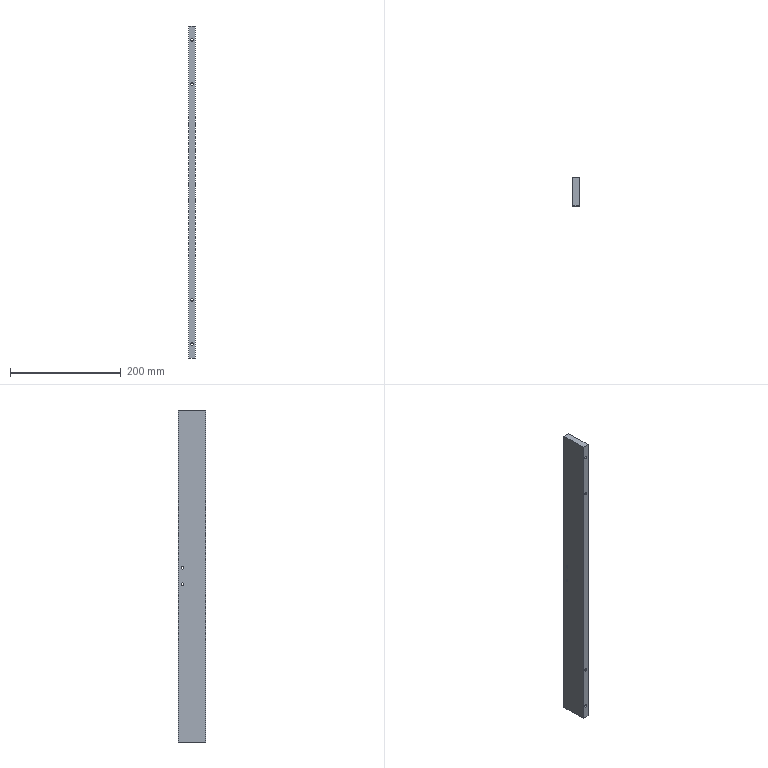Component | SolidWorks | SupportPlate-2 | 1 solid | 18 faces | box 12 x 50 x 600 mm | volume 355602 mm3 | cylinder 12 | plane 6 | commonest cylinder face diameters 5 x12
build123d program:
from build123d import *

# Parameters (mm, degrees)
SKETCH1_W             = 12
SKETCH1_H             = 50
EXTRUDE1_DEPTH        = 600
M6_TAPPED_HOLE1_D     = 5
M6_TAPPED_HOLE2_D     = 5
M6_TAPPED_HOLE2_DEPTH = 15
M6_TAPPED_HOLE2_TIP   = 1.502


with BuildPart() as part:
    # Sketch1 → Extrude1 (new body)
    with BuildSketch(Plane.XY):
        with Locations((49.859, -11.771)):
            Rectangle(SKETCH1_W, SKETCH1_H)
    extrude(amount=EXTRUDE1_DEPTH)

    # M6 Tapped Hole1 (through all)
    with Locations(Plane(origin=(0, 13.229, 0), x_dir=(-1, 0, 0), z_dir=(0, 1, 0))):
        with Locations((-49.859, 25), (-49.859, 105), (-49.859, 575), (-49.859, 495)):
            Hole(M6_TAPPED_HOLE1_D / 2)

    # M6 Tapped Hole2
    with Locations(Plane.ZY.offset(-43.859)):
        with Locations((315, 5.229), (285, 5.229)):
            Hole(M6_TAPPED_HOLE2_D / 2, depth=M6_TAPPED_HOLE2_DEPTH)
            with Locations((0, 0, -(M6_TAPPED_HOLE2_DEPTH + M6_TAPPED_HOLE2_TIP / 2))):  # 118° drill point
                Cone(0, M6_TAPPED_HOLE2_D / 2, M6_TAPPED_HOLE2_TIP, mode=Mode.SUBTRACT)


solid = part.part

# Placed as in the assembly
solid = solid.moved(Location((4.357, 407.754, -296), (0, 0, 0)))
STEP:
#1=COLOUR_RGB('',0.7922,0.8196,0.9333);
#2=FILL_AREA_STYLE_COLOUR('',#1);
#3=FILL_AREA_STYLE('',(#2));
#4=SURFACE_STYLE_FILL_AREA(#3);
#5=SURFACE_SIDE_STYLE('',(#4));
#6=SURFACE_STYLE_USAGE(.BOTH.,#5);
#7=PRESENTATION_STYLE_ASSIGNMENT((#6));
#8=CARTESIAN_POINT('',(2.371,16.259,0.6496));
#9=VERTEX_POINT('',#8);
#10=CARTESIAN_POINT('',(2.371,16.259,0.8465));
#11=VERTEX_POINT('',#10);
#12=CARTESIAN_POINT('',(2.371,16.259,0.748));
#13=DIRECTION('',(-1.,-0.,0.));
#14=DIRECTION('',(0.,-1.,0.));
#15=AXIS2_PLACEMENT_3D('',#12,#13,#14);
#16=CIRCLE('',#15,0.09843);
#17=EDGE_CURVE('',#9,#11,#16,.T.);
#18=ORIENTED_EDGE('',*,*,#17,.F.);
#19=CARTESIAN_POINT('',(1.898,16.259,0.6496));
#20=VERTEX_POINT('',#19);
#21=CARTESIAN_POINT('',(1.898,16.259,0.6496));
#22=DIRECTION('',(-1.,0.,0.));
#23=VECTOR('',#22,39.37);
#24=LINE('',#21,#23);
#25=EDGE_CURVE('',#9,#20,#24,.T.);
#26=ORIENTED_EDGE('',*,*,#25,.T.);
#27=CARTESIAN_POINT('',(1.898,16.259,0.8465));
#28=VERTEX_POINT('',#27);
#29=CARTESIAN_POINT('',(1.898,16.259,0.748));
#30=DIRECTION('',(-1.,0.,0.));
#31=DIRECTION('',(0.,0.,1.));
#32=AXIS2_PLACEMENT_3D('',#29,#30,#31);
#33=CIRCLE('',#32,0.09843);
#34=EDGE_CURVE('',#20,#28,#33,.T.);
#35=ORIENTED_EDGE('',*,*,#34,.T.);
#36=CARTESIAN_POINT('',(1.898,16.259,0.8465));
#37=DIRECTION('',(-1.,0.,0.));
#38=VECTOR('',#37,39.37);
#39=LINE('',#36,#38);
#40=EDGE_CURVE('',#11,#28,#39,.T.);
#41=ORIENTED_EDGE('',*,*,#40,.F.);
#42=EDGE_LOOP('',(#18,#26,#35,#41));
#43=FACE_OUTER_BOUND('',#42,.T.);
#44=CARTESIAN_POINT('',(1.898,16.259,0.748));
#45=DIRECTION('',(-1.,0.,0.));
#46=DIRECTION('',(0.,0.,1.));
#47=AXIS2_PLACEMENT_3D('',#44,#45,#46);
#48=CYLINDRICAL_SURFACE('',#47,0.09843);
#49=ADVANCED_FACE('',(#43),#48,.F.);
#50=CARTESIAN_POINT('',(2.371,16.259,-0.5315));
#51=VERTEX_POINT('',#50);
#52=CARTESIAN_POINT('',(2.371,16.259,-0.3346));
#53=VERTEX_POINT('',#52);
#54=CARTESIAN_POINT('',(2.371,16.259,-0.4331));
#55=DIRECTION('',(-1.,-0.,0.));
#56=DIRECTION('',(0.,-1.,0.));
#57=AXIS2_PLACEMENT_3D('',#54,#55,#56);
#58=CIRCLE('',#57,0.09843);
#59=EDGE_CURVE('',#51,#53,#58,.T.);
#60=ORIENTED_EDGE('',*,*,#59,.F.);
#61=CARTESIAN_POINT('',(1.898,16.259,-0.5315));
#62=VERTEX_POINT('',#61);
#63=CARTESIAN_POINT('',(1.898,16.259,-0.5315));
#64=DIRECTION('',(-1.,0.,0.));
#65=VECTOR('',#64,39.37);
#66=LINE('',#63,#65);
#67=EDGE_CURVE('',#51,#62,#66,.T.);
#68=ORIENTED_EDGE('',*,*,#67,.T.);
#69=CARTESIAN_POINT('',(1.898,16.259,-0.3346));
#70=VERTEX_POINT('',#69);
#71=CARTESIAN_POINT('',(1.898,16.259,-0.4331));
#72=DIRECTION('',(-1.,0.,0.));
#73=DIRECTION('',(0.,0.,1.));
#74=AXIS2_PLACEMENT_3D('',#71,#72,#73);
#75=CIRCLE('',#74,0.09843);
#76=EDGE_CURVE('',#62,#70,#75,.T.);
#77=ORIENTED_EDGE('',*,*,#76,.T.);
#78=CARTESIAN_POINT('',(1.898,16.259,-0.3346));
#79=DIRECTION('',(-1.,0.,0.));
#80=VECTOR('',#79,39.37);
#81=LINE('',#78,#80);
#82=EDGE_CURVE('',#53,#70,#81,.T.);
#83=ORIENTED_EDGE('',*,*,#82,.F.);
#84=EDGE_LOOP('',(#60,#68,#77,#83));
#85=FACE_OUTER_BOUND('',#84,.T.);
#86=CARTESIAN_POINT('',(1.898,16.259,-0.4331));
#87=DIRECTION('',(-1.,0.,0.));
#88=DIRECTION('',(0.,0.,1.));
#89=AXIS2_PLACEMENT_3D('',#86,#87,#88);
#90=CYLINDRICAL_SURFACE('',#89,0.09843);
#91=ADVANCED_FACE('',(#85),#90,.F.);
#92=CARTESIAN_POINT('',(2.134,14.606,-10.768));
#93=VERTEX_POINT('',#92);
#94=CARTESIAN_POINT('',(2.134,14.606,-10.571));
#95=VERTEX_POINT('',#94);
#96=CARTESIAN_POINT('',(2.134,14.606,-10.669));
#97=DIRECTION('',(0.,1.,0.));
#98=DIRECTION('',(0.,0.,1.));
#99=AXIS2_PLACEMENT_3D('',#96,#97,#98);
#100=CIRCLE('',#99,0.09843);
#101=EDGE_CURVE('',#93,#95,#100,.T.);
#102=ORIENTED_EDGE('',*,*,#101,.F.);
#103=CARTESIAN_POINT('',(2.134,16.574,-10.768));
#104=VERTEX_POINT('',#103);
#105=CARTESIAN_POINT('',(2.134,16.574,-10.768));
#106=DIRECTION('',(0.,1.,0.));
#107=VECTOR('',#106,39.37);
#108=LINE('',#105,#107);
#109=EDGE_CURVE('',#93,#104,#108,.T.);
#110=ORIENTED_EDGE('',*,*,#109,.T.);
#111=CARTESIAN_POINT('',(2.134,16.574,-10.571));
#112=VERTEX_POINT('',#111);
#113=CARTESIAN_POINT('',(2.134,16.574,-10.669));
#114=DIRECTION('',(0.,1.,0.));
#115=DIRECTION('',(0.,0.,1.));
#116=AXIS2_PLACEMENT_3D('',#113,#114,#115);
#117=CIRCLE('',#116,0.09843);
#118=EDGE_CURVE('',#104,#112,#117,.T.);
#119=ORIENTED_EDGE('',*,*,#118,.T.);
#120=CARTESIAN_POINT('',(2.134,16.574,-10.571));
#121=DIRECTION('',(0.,1.,0.));
#122=VECTOR('',#121,39.37);
#123=LINE('',#120,#122);
#124=EDGE_CURVE('',#95,#112,#123,.T.);
#125=ORIENTED_EDGE('',*,*,#124,.F.);
#126=EDGE_LOOP('',(#102,#110,#119,#125));
#127=FACE_OUTER_BOUND('',#126,.T.);
#128=CARTESIAN_POINT('',(2.134,16.574,-10.669));
#129=DIRECTION('',(0.,1.,0.));
#130=DIRECTION('',(0.,0.,1.));
#131=AXIS2_PLACEMENT_3D('',#128,#129,#130);
#132=CYLINDRICAL_SURFACE('',#131,0.09843);
#133=ADVANCED_FACE('',(#127),#132,.F.);
#134=CARTESIAN_POINT('',(2.134,14.606,-7.618));
#135=VERTEX_POINT('',#134);
#136=CARTESIAN_POINT('',(2.134,14.606,-7.421));
#137=VERTEX_POINT('',#136);
#138=CARTESIAN_POINT('',(2.134,14.606,-7.52));
#139=DIRECTION('',(0.,1.,0.));
#140=DIRECTION('',(0.,0.,1.));
#141=AXIS2_PLACEMENT_3D('',#138,#139,#140);
#142=CIRCLE('',#141,0.09843);
#143=EDGE_CURVE('',#135,#137,#142,.T.);
#144=ORIENTED_EDGE('',*,*,#143,.F.);
#145=CARTESIAN_POINT('',(2.134,16.574,-7.618));
#146=VERTEX_POINT('',#145);
#147=CARTESIAN_POINT('',(2.134,16.574,-7.618));
#148=DIRECTION('',(0.,1.,0.));
#149=VECTOR('',#148,39.37);
#150=LINE('',#147,#149);
#151=EDGE_CURVE('',#135,#146,#150,.T.);
#152=ORIENTED_EDGE('',*,*,#151,.T.);
#153=CARTESIAN_POINT('',(2.134,16.574,-7.421));
#154=VERTEX_POINT('',#153);
#155=CARTESIAN_POINT('',(2.134,16.574,-7.52));
#156=DIRECTION('',(0.,1.,0.));
#157=DIRECTION('',(0.,0.,1.));
#158=AXIS2_PLACEMENT_3D('',#155,#156,#157);
#159=CIRCLE('',#158,0.09843);
#160=EDGE_CURVE('',#146,#154,#159,.T.);
#161=ORIENTED_EDGE('',*,*,#160,.T.);
#162=CARTESIAN_POINT('',(2.134,16.574,-7.421));
#163=DIRECTION('',(0.,1.,0.));
#164=VECTOR('',#163,39.37);
#165=LINE('',#162,#164);
#166=EDGE_CURVE('',#137,#154,#165,.T.);
#167=ORIENTED_EDGE('',*,*,#166,.F.);
#168=EDGE_LOOP('',(#144,#152,#161,#167));
#169=FACE_OUTER_BOUND('',#168,.T.);
#170=CARTESIAN_POINT('',(2.134,16.574,-7.52));
#171=DIRECTION('',(0.,1.,0.));
#172=DIRECTION('',(0.,0.,1.));
#173=AXIS2_PLACEMENT_3D('',#170,#171,#172);
#174=CYLINDRICAL_SURFACE('',#173,0.09843);
#175=ADVANCED_FACE('',(#169),#174,.F.);
#176=CARTESIAN_POINT('',(2.134,14.606,10.886));
#177=VERTEX_POINT('',#176);
#178=CARTESIAN_POINT('',(2.134,14.606,11.083));
#179=VERTEX_POINT('',#178);
#180=CARTESIAN_POINT('',(2.134,14.606,10.984));
#181=DIRECTION('',(0.,1.,0.));
#182=DIRECTION('',(0.,0.,1.));
#183=AXIS2_PLACEMENT_3D('',#180,#181,#182);
#184=CIRCLE('',#183,0.09843);
#185=EDGE_CURVE('',#177,#179,#184,.T.);
#186=ORIENTED_EDGE('',*,*,#185,.F.);
#187=CARTESIAN_POINT('',(2.134,16.574,10.886));
#188=VERTEX_POINT('',#187);
#189=CARTESIAN_POINT('',(2.134,16.574,10.886));
#190=DIRECTION('',(0.,1.,0.));
#191=VECTOR('',#190,39.37);
#192=LINE('',#189,#191);
#193=EDGE_CURVE('',#177,#188,#192,.T.);
#194=ORIENTED_EDGE('',*,*,#193,.T.);
#195=CARTESIAN_POINT('',(2.134,16.574,11.083));
#196=VERTEX_POINT('',#195);
#197=CARTESIAN_POINT('',(2.134,16.574,10.984));
#198=DIRECTION('',(0.,1.,0.));
#199=DIRECTION('',(0.,0.,1.));
#200=AXIS2_PLACEMENT_3D('',#197,#198,#199);
#201=CIRCLE('',#200,0.09843);
#202=EDGE_CURVE('',#188,#196,#201,.T.);
#203=ORIENTED_EDGE('',*,*,#202,.T.);
#204=CARTESIAN_POINT('',(2.134,16.574,11.083));
#205=DIRECTION('',(0.,1.,0.));
#206=VECTOR('',#205,39.37);
#207=LINE('',#204,#206);
#208=EDGE_CURVE('',#179,#196,#207,.T.);
#209=ORIENTED_EDGE('',*,*,#208,.F.);
#210=EDGE_LOOP('',(#186,#194,#203,#209));
#211=FACE_OUTER_BOUND('',#210,.T.);
#212=CARTESIAN_POINT('',(2.134,16.574,10.984));
#213=DIRECTION('',(0.,1.,0.));
#214=DIRECTION('',(0.,0.,1.));
#215=AXIS2_PLACEMENT_3D('',#212,#213,#214);
#216=CYLINDRICAL_SURFACE('',#215,0.09843);
#217=ADVANCED_FACE('',(#211),#216,.F.);
#218=CARTESIAN_POINT('',(2.134,14.606,7.736));
#219=VERTEX_POINT('',#218);
#220=CARTESIAN_POINT('',(2.134,14.606,7.933));
#221=VERTEX_POINT('',#220);
#222=CARTESIAN_POINT('',(2.134,14.606,7.835));
#223=DIRECTION('',(0.,1.,0.));
#224=DIRECTION('',(0.,0.,1.));
#225=AXIS2_PLACEMENT_3D('',#222,#223,#224);
#226=CIRCLE('',#225,0.09843);
#227=EDGE_CURVE('',#219,#221,#226,.T.);
#228=ORIENTED_EDGE('',*,*,#227,.F.);
#229=CARTESIAN_POINT('',(2.134,16.574,7.736));
#230=VERTEX_POINT('',#229);
#231=CARTESIAN_POINT('',(2.134,16.574,7.736));
#232=DIRECTION('',(0.,1.,0.));
#233=VECTOR('',#232,39.37);
#234=LINE('',#231,#233);
#235=EDGE_CURVE('',#219,#230,#234,.T.);
#236=ORIENTED_EDGE('',*,*,#235,.T.);
#237=CARTESIAN_POINT('',(2.134,16.574,7.933));
#238=VERTEX_POINT('',#237);
#239=CARTESIAN_POINT('',(2.134,16.574,7.835));
#240=DIRECTION('',(0.,1.,0.));
#241=DIRECTION('',(0.,0.,1.));
#242=AXIS2_PLACEMENT_3D('',#239,#240,#241);
#243=CIRCLE('',#242,0.09843);
#244=EDGE_CURVE('',#230,#238,#243,.T.);
#245=ORIENTED_EDGE('',*,*,#244,.T.);
#246=CARTESIAN_POINT('',(2.134,16.574,7.933));
#247=DIRECTION('',(0.,1.,0.));
#248=VECTOR('',#247,39.37);
#249=LINE('',#246,#248);
#250=EDGE_CURVE('',#221,#238,#249,.T.);
#251=ORIENTED_EDGE('',*,*,#250,.F.);
#252=EDGE_LOOP('',(#228,#236,#245,#251));
#253=FACE_OUTER_BOUND('',#252,.T.);
#254=CARTESIAN_POINT('',(2.134,16.574,7.835));
#255=DIRECTION('',(0.,1.,0.));
#256=DIRECTION('',(0.,0.,1.));
#257=AXIS2_PLACEMENT_3D('',#254,#255,#256);
#258=CYLINDRICAL_SURFACE('',#257,0.09843);
#259=ADVANCED_FACE('',(#253),#258,.F.);
#260=CARTESIAN_POINT('',(1.898,16.259,0.748));
#261=DIRECTION('',(-1.,0.,0.));
#262=DIRECTION('',(0.,0.,1.));
#263=AXIS2_PLACEMENT_3D('',#260,#261,#262);
#264=CIRCLE('',#263,0.09843);
#265=EDGE_CURVE('',#28,#20,#264,.T.);
#266=ORIENTED_EDGE('',*,*,#265,.F.);
#267=ORIENTED_EDGE('',*,*,#34,.F.);
#268=EDGE_LOOP('',(#266,#267));
#269=FACE_BOUND('',#268,.T.);
#270=CARTESIAN_POINT('',(1.898,16.259,-0.4331));
#271=DIRECTION('',(-1.,0.,0.));
#272=DIRECTION('',(0.,0.,1.));
#273=AXIS2_PLACEMENT_3D('',#270,#271,#272);
#274=CIRCLE('',#273,0.09843);
#275=EDGE_CURVE('',#70,#62,#274,.T.);
#276=ORIENTED_EDGE('',*,*,#275,.F.);
#277=ORIENTED_EDGE('',*,*,#76,.F.);
#278=EDGE_LOOP('',(#276,#277));
#279=FACE_BOUND('',#278,.T.);
#280=CARTESIAN_POINT('',(1.898,16.574,-11.654));
#281=VERTEX_POINT('',#280);
#282=CARTESIAN_POINT('',(1.898,14.606,-11.654));
#283=VERTEX_POINT('',#282);
#284=CARTESIAN_POINT('',(1.898,16.574,-11.654));
#285=DIRECTION('',(0.,-1.,0.));
#286=VECTOR('',#285,39.37);
#287=LINE('',#284,#286);
#288=EDGE_CURVE('',#281,#283,#287,.T.);
#289=ORIENTED_EDGE('',*,*,#288,.T.);
#290=CARTESIAN_POINT('',(1.898,14.606,11.969));
#291=VERTEX_POINT('',#290);
#292=CARTESIAN_POINT('',(1.898,14.606,11.969));
#293=DIRECTION('',(0.,0.,-1.));
#294=VECTOR('',#293,39.37);
#295=LINE('',#292,#294);
#296=EDGE_CURVE('',#291,#283,#295,.T.);
#297=ORIENTED_EDGE('',*,*,#296,.F.);
#298=CARTESIAN_POINT('',(1.898,16.574,11.969));
#299=VERTEX_POINT('',#298);
#300=CARTESIAN_POINT('',(1.898,16.574,11.969));
#301=DIRECTION('',(0.,-1.,0.));
#302=VECTOR('',#301,39.37);
#303=LINE('',#300,#302);
#304=EDGE_CURVE('',#299,#291,#303,.T.);
#305=ORIENTED_EDGE('',*,*,#304,.F.);
#306=CARTESIAN_POINT('',(1.898,16.574,11.969));
#307=DIRECTION('',(0.,0.,-1.));
#308=VECTOR('',#307,39.37);
#309=LINE('',#306,#308);
#310=EDGE_CURVE('',#299,#281,#309,.T.);
#311=ORIENTED_EDGE('',*,*,#310,.T.);
#312=EDGE_LOOP('',(#289,#297,#305,#311));
#313=FACE_OUTER_BOUND('',#312,.T.);
#314=CARTESIAN_POINT('',(1.898,16.574,11.969));
#315=DIRECTION('',(1.,0.,0.));
#316=DIRECTION('',(0.,0.,-1.));
#317=AXIS2_PLACEMENT_3D('',#314,#315,#316);
#318=PLANE('',#317);
#319=ADVANCED_FACE('',(#269,#279,#313),#318,.F.);
#320=CARTESIAN_POINT('',(2.134,14.606,-10.669));
#321=DIRECTION('',(0.,1.,0.));
#322=DIRECTION('',(0.,0.,1.));
#323=AXIS2_PLACEMENT_3D('',#320,#321,#322);
#324=CIRCLE('',#323,0.09843);
#325=EDGE_CURVE('',#95,#93,#324,.T.);
#326=ORIENTED_EDGE('',*,*,#325,.T.);
#327=ORIENTED_EDGE('',*,*,#101,.T.);
#328=EDGE_LOOP('',(#326,#327));
#329=FACE_BOUND('',#328,.T.);
#330=CARTESIAN_POINT('',(2.134,14.606,-7.52));
#331=DIRECTION('',(0.,1.,0.));
#332=DIRECTION('',(0.,0.,1.));
#333=AXIS2_PLACEMENT_3D('',#330,#331,#332);
#334=CIRCLE('',#333,0.09843);
#335=EDGE_CURVE('',#137,#135,#334,.T.);
#336=ORIENTED_EDGE('',*,*,#335,.T.);
#337=ORIENTED_EDGE('',*,*,#143,.T.);
#338=EDGE_LOOP('',(#336,#337));
#339=FACE_BOUND('',#338,.T.);
#340=CARTESIAN_POINT('',(2.134,14.606,10.984));
#341=DIRECTION('',(0.,1.,0.));
#342=DIRECTION('',(0.,0.,1.));
#343=AXIS2_PLACEMENT_3D('',#340,#341,#342);
#344=CIRCLE('',#343,0.09843);
#345=EDGE_CURVE('',#179,#177,#344,.T.);
#346=ORIENTED_EDGE('',*,*,#345,.T.);
#347=ORIENTED_EDGE('',*,*,#185,.T.);
#348=EDGE_LOOP('',(#346,#347));
#349=FACE_BOUND('',#348,.T.);
#350=CARTESIAN_POINT('',(2.134,14.606,7.835));
#351=DIRECTION('',(0.,1.,0.));
#352=DIRECTION('',(0.,0.,1.));
#353=AXIS2_PLACEMENT_3D('',#350,#351,#352);
#354=CIRCLE('',#353,0.09843);
#355=EDGE_CURVE('',#221,#219,#354,.T.);
#356=ORIENTED_EDGE('',*,*,#355,.T.);
#357=ORIENTED_EDGE('',*,*,#227,.T.);
#358=EDGE_LOOP('',(#356,#357));
#359=FACE_BOUND('',#358,.T.);
#360=CARTESIAN_POINT('',(2.371,14.606,-11.654));
#361=VERTEX_POINT('',#360);
#362=CARTESIAN_POINT('',(1.898,14.606,-11.654));
#363=DIRECTION('',(1.,0.,0.));
#364=VECTOR('',#363,39.37);
#365=LINE('',#362,#364);
#366=EDGE_CURVE('',#283,#361,#365,.T.);
#367=ORIENTED_EDGE('',*,*,#366,.T.);
#368=CARTESIAN_POINT('',(2.371,14.606,11.969));
#369=VERTEX_POINT('',#368);
#370=CARTESIAN_POINT('',(2.371,14.606,11.969));
#371=DIRECTION('',(0.,0.,-1.));
#372=VECTOR('',#371,39.37);
#373=LINE('',#370,#372);
#374=EDGE_CURVE('',#369,#361,#373,.T.);
#375=ORIENTED_EDGE('',*,*,#374,.F.);
#376=CARTESIAN_POINT('',(1.898,14.606,11.969));
#377=DIRECTION('',(1.,0.,0.));
#378=VECTOR('',#377,39.37);
#379=LINE('',#376,#378);
#380=EDGE_CURVE('',#291,#369,#379,.T.);
#381=ORIENTED_EDGE('',*,*,#380,.F.);
#382=ORIENTED_EDGE('',*,*,#296,.T.);
#383=EDGE_LOOP('',(#367,#375,#381,#382));
#384=FACE_OUTER_BOUND('',#383,.T.);
#385=CARTESIAN_POINT('',(1.898,14.606,11.969));
#386=DIRECTION('',(0.,1.,0.));
#387=DIRECTION('',(0.,0.,1.));
#388=AXIS2_PLACEMENT_3D('',#385,#386,#387);
#389=PLANE('',#388);
#390=ADVANCED_FACE('',(#329,#339,#349,#359,#384),#389,.F.);
#391=CARTESIAN_POINT('',(2.371,16.259,0.748));
#392=DIRECTION('',(-1.,-0.,0.));
#393=DIRECTION('',(0.,-1.,0.));
#394=AXIS2_PLACEMENT_3D('',#391,#392,#393);
#395=CIRCLE('',#394,0.09843);
#396=EDGE_CURVE('',#11,#9,#395,.T.);
#397=ORIENTED_EDGE('',*,*,#396,.T.);
#398=ORIENTED_EDGE('',*,*,#17,.T.);
#399=EDGE_LOOP('',(#397,#398));
#400=FACE_BOUND('',#399,.T.);
#401=CARTESIAN_POINT('',(2.371,16.259,-0.4331));
#402=DIRECTION('',(-1.,-0.,0.));
#403=DIRECTION('',(0.,-1.,0.));
#404=AXIS2_PLACEMENT_3D('',#401,#402,#403);
#405=CIRCLE('',#404,0.09843);
#406=EDGE_CURVE('',#53,#51,#405,.T.);
#407=ORIENTED_EDGE('',*,*,#406,.T.);
#408=ORIENTED_EDGE('',*,*,#59,.T.);
#409=EDGE_LOOP('',(#407,#408));
#410=FACE_BOUND('',#409,.T.);
#411=CARTESIAN_POINT('',(2.371,16.574,-11.654));
#412=VERTEX_POINT('',#411);
#413=CARTESIAN_POINT('',(2.371,16.574,-11.654));
#414=DIRECTION('',(-0.,1.,0.));
#415=VECTOR('',#414,39.37);
#416=LINE('',#413,#415);
#417=EDGE_CURVE('',#361,#412,#416,.T.);
#418=ORIENTED_EDGE('',*,*,#417,.T.);
#419=CARTESIAN_POINT('',(2.371,16.574,11.969));
#420=VERTEX_POINT('',#419);
#421=CARTESIAN_POINT('',(2.371,16.574,11.969));
#422=DIRECTION('',(0.,0.,-1.));
#423=VECTOR('',#422,39.37);
#424=LINE('',#421,#423);
#425=EDGE_CURVE('',#420,#412,#424,.T.);
#426=ORIENTED_EDGE('',*,*,#425,.F.);
#427=CARTESIAN_POINT('',(2.371,16.574,11.969));
#428=DIRECTION('',(-0.,1.,0.));
#429=VECTOR('',#428,39.37);
#430=LINE('',#427,#429);
#431=EDGE_CURVE('',#369,#420,#430,.T.);
#432=ORIENTED_EDGE('',*,*,#431,.F.);
#433=ORIENTED_EDGE('',*,*,#374,.T.);
#434=EDGE_LOOP('',(#418,#426,#432,#433));
#435=FACE_OUTER_BOUND('',#434,.T.);
#436=CARTESIAN_POINT('',(2.371,16.574,11.969));
#437=DIRECTION('',(-1.,-0.,0.));
#438=DIRECTION('',(0.,-1.,0.));
#439=AXIS2_PLACEMENT_3D('',#436,#437,#438);
#440=PLANE('',#439);
#441=ADVANCED_FACE('',(#400,#410,#435),#440,.F.);
#442=CARTESIAN_POINT('',(2.134,16.574,-10.669));
#443=DIRECTION('',(0.,1.,0.));
#444=DIRECTION('',(0.,0.,1.));
#445=AXIS2_PLACEMENT_3D('',#442,#443,#444);
#446=CIRCLE('',#445,0.09843);
#447=EDGE_CURVE('',#112,#104,#446,.T.);
#448=ORIENTED_EDGE('',*,*,#447,.F.);
#449=ORIENTED_EDGE('',*,*,#118,.F.);
#450=EDGE_LOOP('',(#448,#449));
#451=FACE_BOUND('',#450,.T.);
#452=CARTESIAN_POINT('',(2.134,16.574,-7.52));
#453=DIRECTION('',(0.,1.,0.));
#454=DIRECTION('',(0.,0.,1.));
#455=AXIS2_PLACEMENT_3D('',#452,#453,#454);
#456=CIRCLE('',#455,0.09843);
#457=EDGE_CURVE('',#154,#146,#456,.T.);
#458=ORIENTED_EDGE('',*,*,#457,.F.);
#459=ORIENTED_EDGE('',*,*,#160,.F.);
#460=EDGE_LOOP('',(#458,#459));
#461=FACE_BOUND('',#460,.T.);
#462=CARTESIAN_POINT('',(2.134,16.574,10.984));
#463=DIRECTION('',(0.,1.,0.));
#464=DIRECTION('',(0.,0.,1.));
#465=AXIS2_PLACEMENT_3D('',#462,#463,#464);
#466=CIRCLE('',#465,0.09843);
#467=EDGE_CURVE('',#196,#188,#466,.T.);
#468=ORIENTED_EDGE('',*,*,#467,.F.);
#469=ORIENTED_EDGE('',*,*,#202,.F.);
#470=EDGE_LOOP('',(#468,#469));
#471=FACE_BOUND('',#470,.T.);
#472=CARTESIAN_POINT('',(2.134,16.574,7.835));
#473=DIRECTION('',(0.,1.,0.));
#474=DIRECTION('',(0.,0.,1.));
#475=AXIS2_PLACEMENT_3D('',#472,#473,#474);
#476=CIRCLE('',#475,0.09843);
#477=EDGE_CURVE('',#238,#230,#476,.T.);
#478=ORIENTED_EDGE('',*,*,#477,.F.);
#479=ORIENTED_EDGE('',*,*,#244,.F.);
#480=EDGE_LOOP('',(#478,#479));
#481=FACE_BOUND('',#480,.T.);
#482=CARTESIAN_POINT('',(1.898,16.574,-11.654));
#483=DIRECTION('',(-1.,0.,0.));
#484=VECTOR('',#483,39.37);
#485=LINE('',#482,#484);
#486=EDGE_CURVE('',#412,#281,#485,.T.);
#487=ORIENTED_EDGE('',*,*,#486,.T.);
#488=ORIENTED_EDGE('',*,*,#310,.F.);
#489=CARTESIAN_POINT('',(1.898,16.574,11.969));
#490=DIRECTION('',(-1.,0.,0.));
#491=VECTOR('',#490,39.37);
#492=LINE('',#489,#491);
#493=EDGE_CURVE('',#420,#299,#492,.T.);
#494=ORIENTED_EDGE('',*,*,#493,.F.);
#495=ORIENTED_EDGE('',*,*,#425,.T.);
#496=EDGE_LOOP('',(#487,#488,#494,#495));
#497=FACE_OUTER_BOUND('',#496,.T.);
#498=CARTESIAN_POINT('',(1.898,16.574,11.969));
#499=DIRECTION('',(0.,-1.,0.));
#500=DIRECTION('',(0.,0.,-1.));
#501=AXIS2_PLACEMENT_3D('',#498,#499,#500);
#502=PLANE('',#501);
#503=ADVANCED_FACE('',(#451,#461,#471,#481,#497),#502,.F.);
#504=ORIENTED_EDGE('',*,*,#304,.T.);
#505=ORIENTED_EDGE('',*,*,#380,.T.);
#506=ORIENTED_EDGE('',*,*,#431,.T.);
#507=ORIENTED_EDGE('',*,*,#493,.T.);
#508=EDGE_LOOP('',(#504,#505,#506,#507));
#509=FACE_OUTER_BOUND('',#508,.T.);
#510=CARTESIAN_POINT('',(1.898,14.606,11.969));
#511=DIRECTION('',(0.,0.,1.));
#512=DIRECTION('',(1.,0.,0.));
#513=AXIS2_PLACEMENT_3D('',#510,#511,#512);
#514=PLANE('',#513);
#515=ADVANCED_FACE('',(#509),#514,.T.);
#516=ORIENTED_EDGE('',*,*,#288,.F.);
#517=ORIENTED_EDGE('',*,*,#486,.F.);
#518=ORIENTED_EDGE('',*,*,#417,.F.);
#519=ORIENTED_EDGE('',*,*,#366,.F.);
#520=EDGE_LOOP('',(#516,#517,#518,#519));
#521=FACE_OUTER_BOUND('',#520,.T.);
#522=CARTESIAN_POINT('',(1.898,14.606,-11.654));
#523=DIRECTION('',(0.,0.,1.));
#524=DIRECTION('',(1.,0.,0.));
#525=AXIS2_PLACEMENT_3D('',#522,#523,#524);
#526=PLANE('',#525);
#527=ADVANCED_FACE('',(#521),#526,.F.);
#528=ORIENTED_EDGE('',*,*,#235,.F.);
#529=ORIENTED_EDGE('',*,*,#355,.F.);
#530=ORIENTED_EDGE('',*,*,#250,.T.);
#531=ORIENTED_EDGE('',*,*,#477,.T.);
#532=EDGE_LOOP('',(#528,#529,#530,#531));
#533=FACE_OUTER_BOUND('',#532,.T.);
#534=CARTESIAN_POINT('',(2.134,16.574,7.835));
#535=DIRECTION('',(0.,1.,0.));
#536=DIRECTION('',(0.,0.,1.));
#537=AXIS2_PLACEMENT_3D('',#534,#535,#536);
#538=CYLINDRICAL_SURFACE('',#537,0.09843);
#539=ADVANCED_FACE('',(#533),#538,.F.);
#540=ORIENTED_EDGE('',*,*,#193,.F.);
#541=ORIENTED_EDGE('',*,*,#345,.F.);
#542=ORIENTED_EDGE('',*,*,#208,.T.);
#543=ORIENTED_EDGE('',*,*,#467,.T.);
#544=EDGE_LOOP('',(#540,#541,#542,#543));
#545=FACE_OUTER_BOUND('',#544,.T.);
#546=CARTESIAN_POINT('',(2.134,16.574,10.984));
#547=DIRECTION('',(0.,1.,0.));
#548=DIRECTION('',(0.,0.,1.));
#549=AXIS2_PLACEMENT_3D('',#546,#547,#548);
#550=CYLINDRICAL_SURFACE('',#549,0.09843);
#551=ADVANCED_FACE('',(#545),#550,.F.);
#552=ORIENTED_EDGE('',*,*,#151,.F.);
#553=ORIENTED_EDGE('',*,*,#335,.F.);
#554=ORIENTED_EDGE('',*,*,#166,.T.);
#555=ORIENTED_EDGE('',*,*,#457,.T.);
#556=EDGE_LOOP('',(#552,#553,#554,#555));
#557=FACE_OUTER_BOUND('',#556,.T.);
#558=CARTESIAN_POINT('',(2.134,16.574,-7.52));
#559=DIRECTION('',(0.,1.,0.));
#560=DIRECTION('',(0.,0.,1.));
#561=AXIS2_PLACEMENT_3D('',#558,#559,#560);
#562=CYLINDRICAL_SURFACE('',#561,0.09843);
#563=ADVANCED_FACE('',(#557),#562,.F.);
#564=ORIENTED_EDGE('',*,*,#109,.F.);
#565=ORIENTED_EDGE('',*,*,#325,.F.);
#566=ORIENTED_EDGE('',*,*,#124,.T.);
#567=ORIENTED_EDGE('',*,*,#447,.T.);
#568=EDGE_LOOP('',(#564,#565,#566,#567));
#569=FACE_OUTER_BOUND('',#568,.T.);
#570=CARTESIAN_POINT('',(2.134,16.574,-10.669));
#571=DIRECTION('',(0.,1.,0.));
#572=DIRECTION('',(0.,0.,1.));
#573=AXIS2_PLACEMENT_3D('',#570,#571,#572);
#574=CYLINDRICAL_SURFACE('',#573,0.09843);
#575=ADVANCED_FACE('',(#569),#574,.F.);
#576=ORIENTED_EDGE('',*,*,#67,.F.);
#577=ORIENTED_EDGE('',*,*,#406,.F.);
#578=ORIENTED_EDGE('',*,*,#82,.T.);
#579=ORIENTED_EDGE('',*,*,#275,.T.);
#580=EDGE_LOOP('',(#576,#577,#578,#579));
#581=FACE_OUTER_BOUND('',#580,.T.);
#582=CARTESIAN_POINT('',(1.898,16.259,-0.4331));
#583=DIRECTION('',(-1.,0.,0.));
#584=DIRECTION('',(0.,0.,1.));
#585=AXIS2_PLACEMENT_3D('',#582,#583,#584);
#586=CYLINDRICAL_SURFACE('',#585,0.09843);
#587=ADVANCED_FACE('',(#581),#586,.F.);
#588=ORIENTED_EDGE('',*,*,#25,.F.);
#589=ORIENTED_EDGE('',*,*,#396,.F.);
#590=ORIENTED_EDGE('',*,*,#40,.T.);
#591=ORIENTED_EDGE('',*,*,#265,.T.);
#592=EDGE_LOOP('',(#588,#589,#590,#591));
#593=FACE_OUTER_BOUND('',#592,.T.);
#594=CARTESIAN_POINT('',(1.898,16.259,0.748));
#595=DIRECTION('',(-1.,0.,0.));
#596=DIRECTION('',(0.,0.,1.));
#597=AXIS2_PLACEMENT_3D('',#594,#595,#596);
#598=CYLINDRICAL_SURFACE('',#597,0.09843);
#599=ADVANCED_FACE('',(#593),#598,.F.);
#600=CLOSED_SHELL('',(#49,#91,#133,#175,#217,#259,#319,#390,#441,#503,#515,#527,#539,#551,#563,#575,#587,#599));
#601=MANIFOLD_SOLID_BREP('',#600);
#602=STYLED_ITEM('',(#7),#601);
#603=(LENGTH_UNIT()NAMED_UNIT(*)SI_UNIT($,.METRE.));
#604=LENGTH_MEASURE_WITH_UNIT(LENGTH_MEASURE(0.0254),#603);
#605=DIMENSIONAL_EXPONENTS(1.,0.,0.,0.,0.,0.,0.);
#606=(CONVERSION_BASED_UNIT('',#604)LENGTH_UNIT()NAMED_UNIT(#605));
#607=UNCERTAINTY_MEASURE_WITH_UNIT(LENGTH_MEASURE(0.00001),#606,'','');
#608=(NAMED_UNIT(*)PLANE_ANGLE_UNIT()SI_UNIT($,.RADIAN.));
#609=(NAMED_UNIT(*)SI_UNIT($,.STERADIAN.)SOLID_ANGLE_UNIT());
#610=(GEOMETRIC_REPRESENTATION_CONTEXT(3)GLOBAL_UNCERTAINTY_ASSIGNED_CONTEXT((#607))GLOBAL_UNIT_ASSIGNED_CONTEXT((#606,#608,#609))REPRESENTATION_CONTEXT('',''));
#611=MECHANICAL_DESIGN_GEOMETRIC_PRESENTATION_REPRESENTATION('',(#602),#610);
#612=PRESENTATION_LAYER_ASSIGNMENT('','',(#602));
#613=CARTESIAN_POINT('',(0.,0.,0.));
#614=DIRECTION('',(0.,0.,1.));
#615=DIRECTION('',(1.,0.,0.));
#616=AXIS2_PLACEMENT_3D('',#613,#614,#615);
#617=(LENGTH_UNIT()NAMED_UNIT(*)SI_UNIT($,.METRE.));
#618=LENGTH_MEASURE_WITH_UNIT(LENGTH_MEASURE(0.0254),#617);
#619=DIMENSIONAL_EXPONENTS(1.,0.,0.,0.,0.,0.,0.);
#620=(CONVERSION_BASED_UNIT('',#618)LENGTH_UNIT()NAMED_UNIT(#619));
#621=UNCERTAINTY_MEASURE_WITH_UNIT(LENGTH_MEASURE(0.00001),#620,'','');
#622=(NAMED_UNIT(*)PLANE_ANGLE_UNIT()SI_UNIT($,.RADIAN.));
#623=(NAMED_UNIT(*)SI_UNIT($,.STERADIAN.)SOLID_ANGLE_UNIT());
#624=(GEOMETRIC_REPRESENTATION_CONTEXT(3)GLOBAL_UNCERTAINTY_ASSIGNED_CONTEXT((#621))GLOBAL_UNIT_ASSIGNED_CONTEXT((#620,#622,#623))REPRESENTATION_CONTEXT('',''));
#625=ADVANCED_BREP_SHAPE_REPRESENTATION('',(#601,#616),#624);